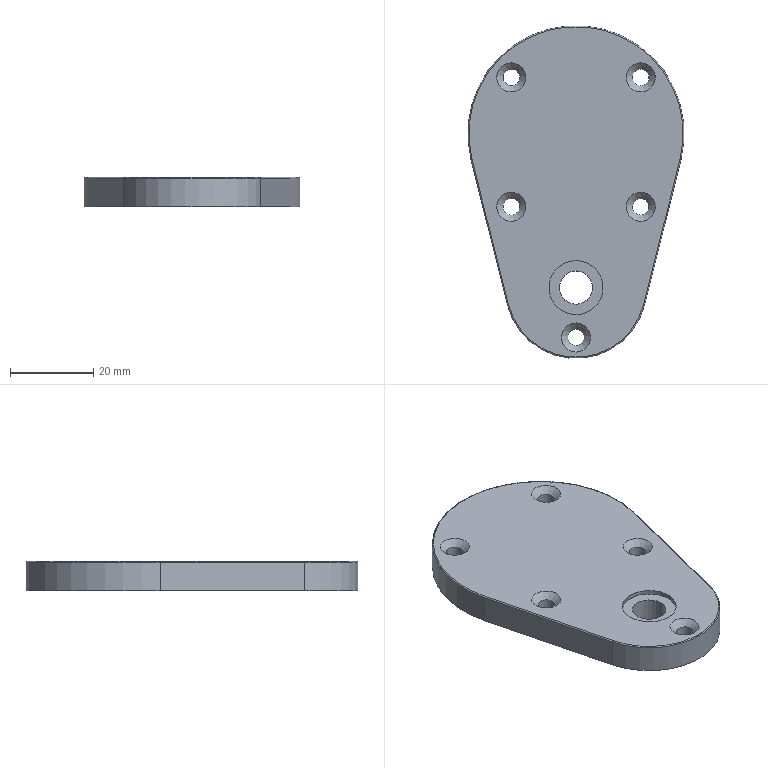Component | NX | TOP_CASING | 1 solid | 23 faces | volume 21114 mm3 | cylinder 11 | plane 5 | cone 5 | torus 2 | commonest cylinder face diameters 4 x5 0.5 x2 34 x1 52 x1 8 x1 13 x1